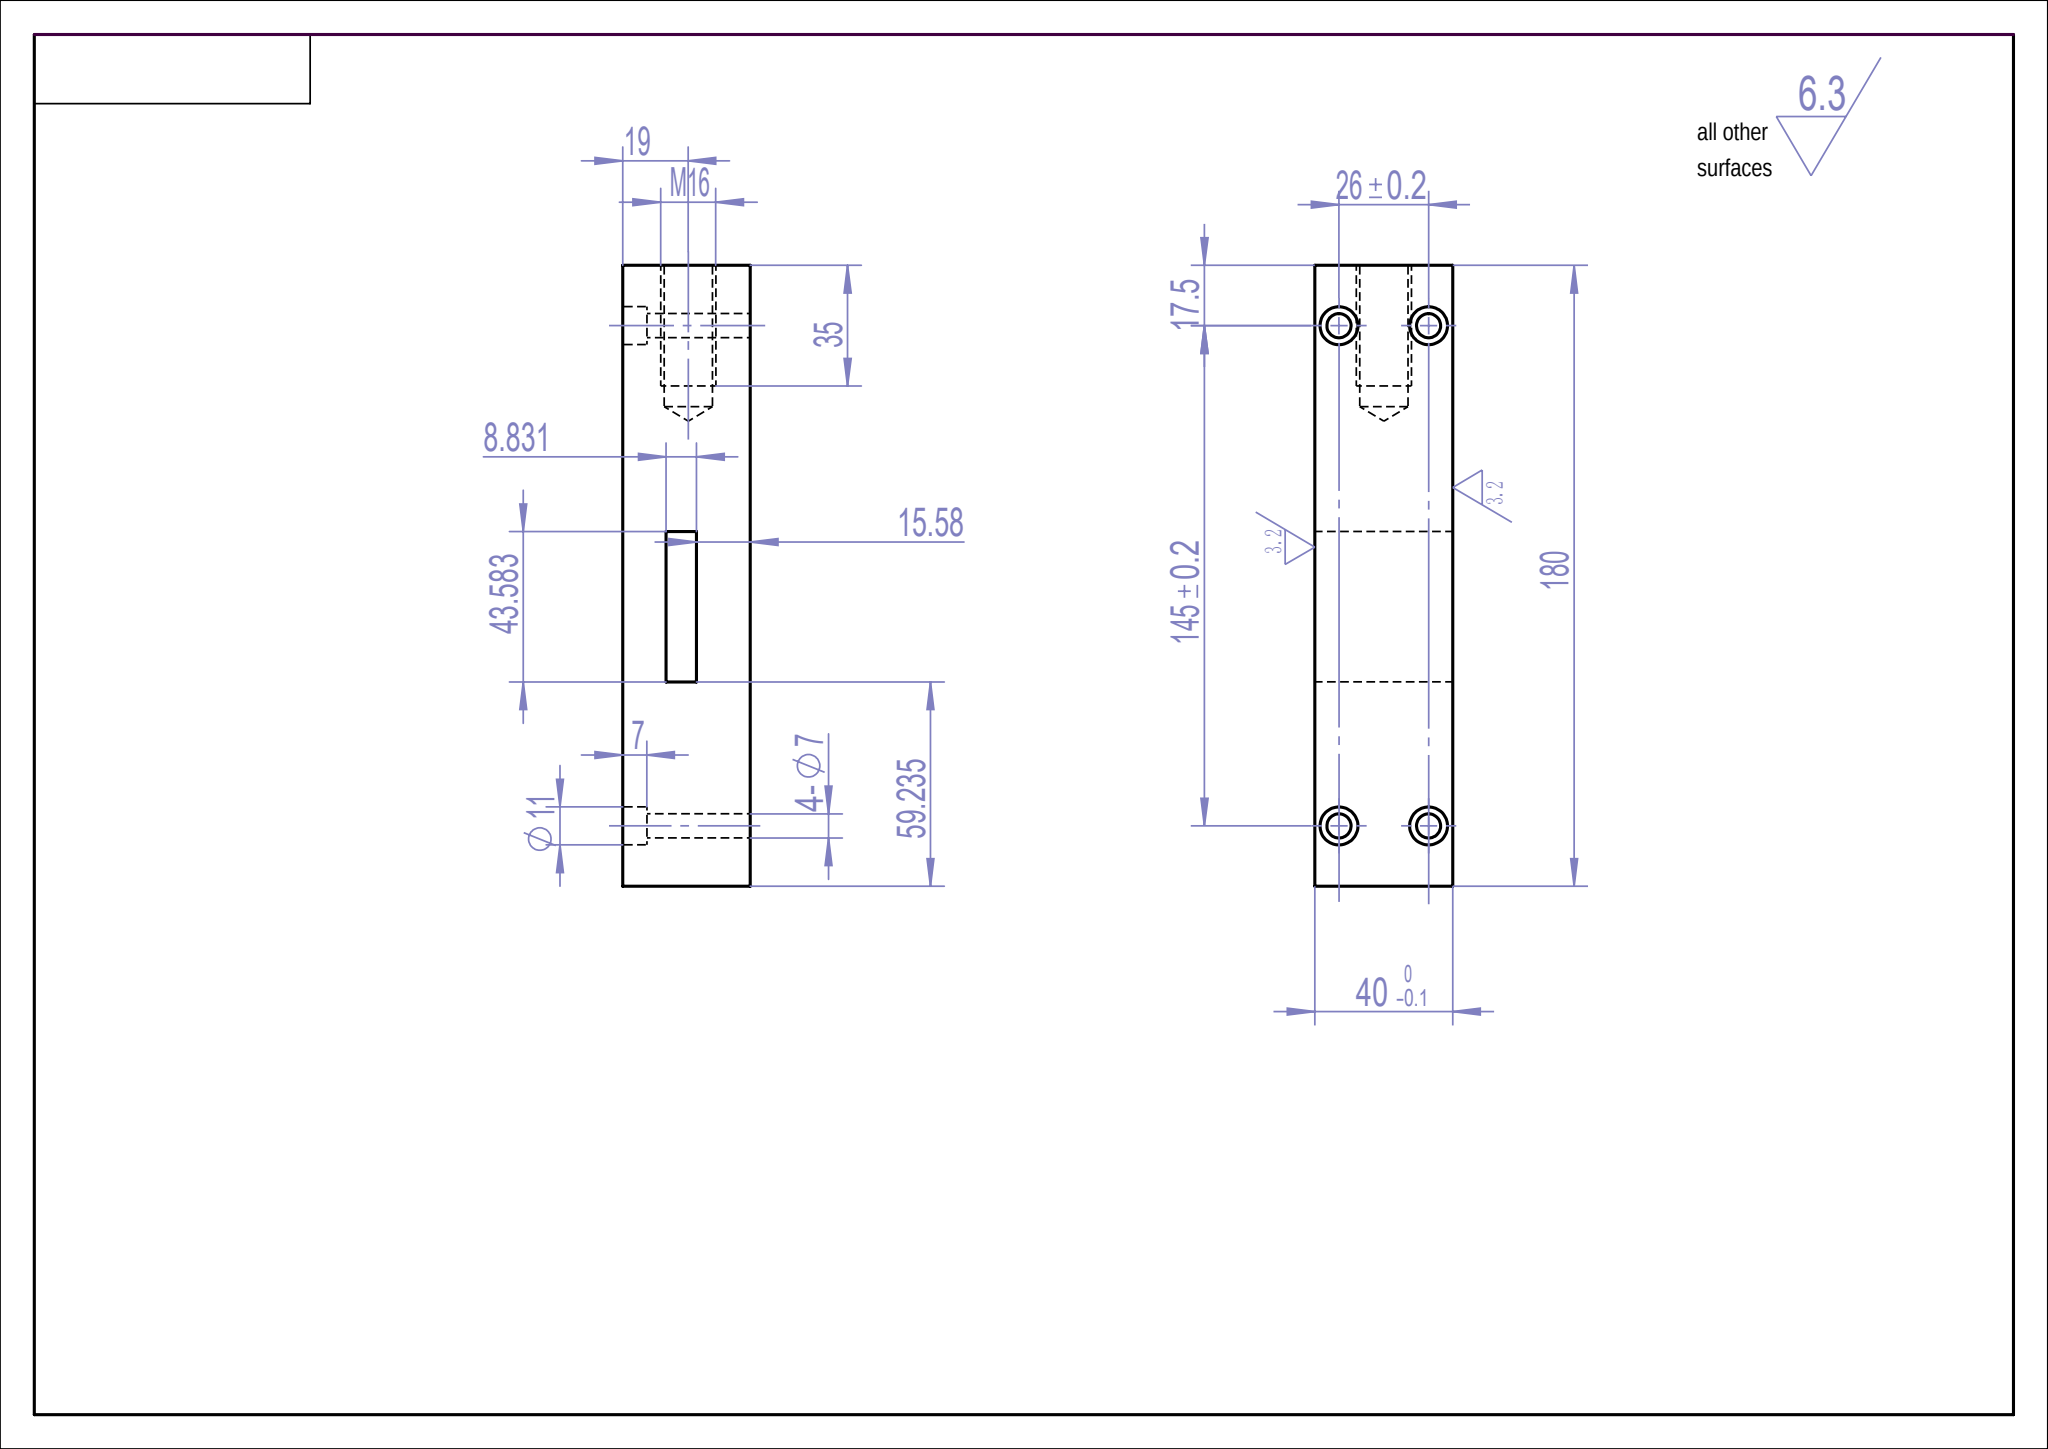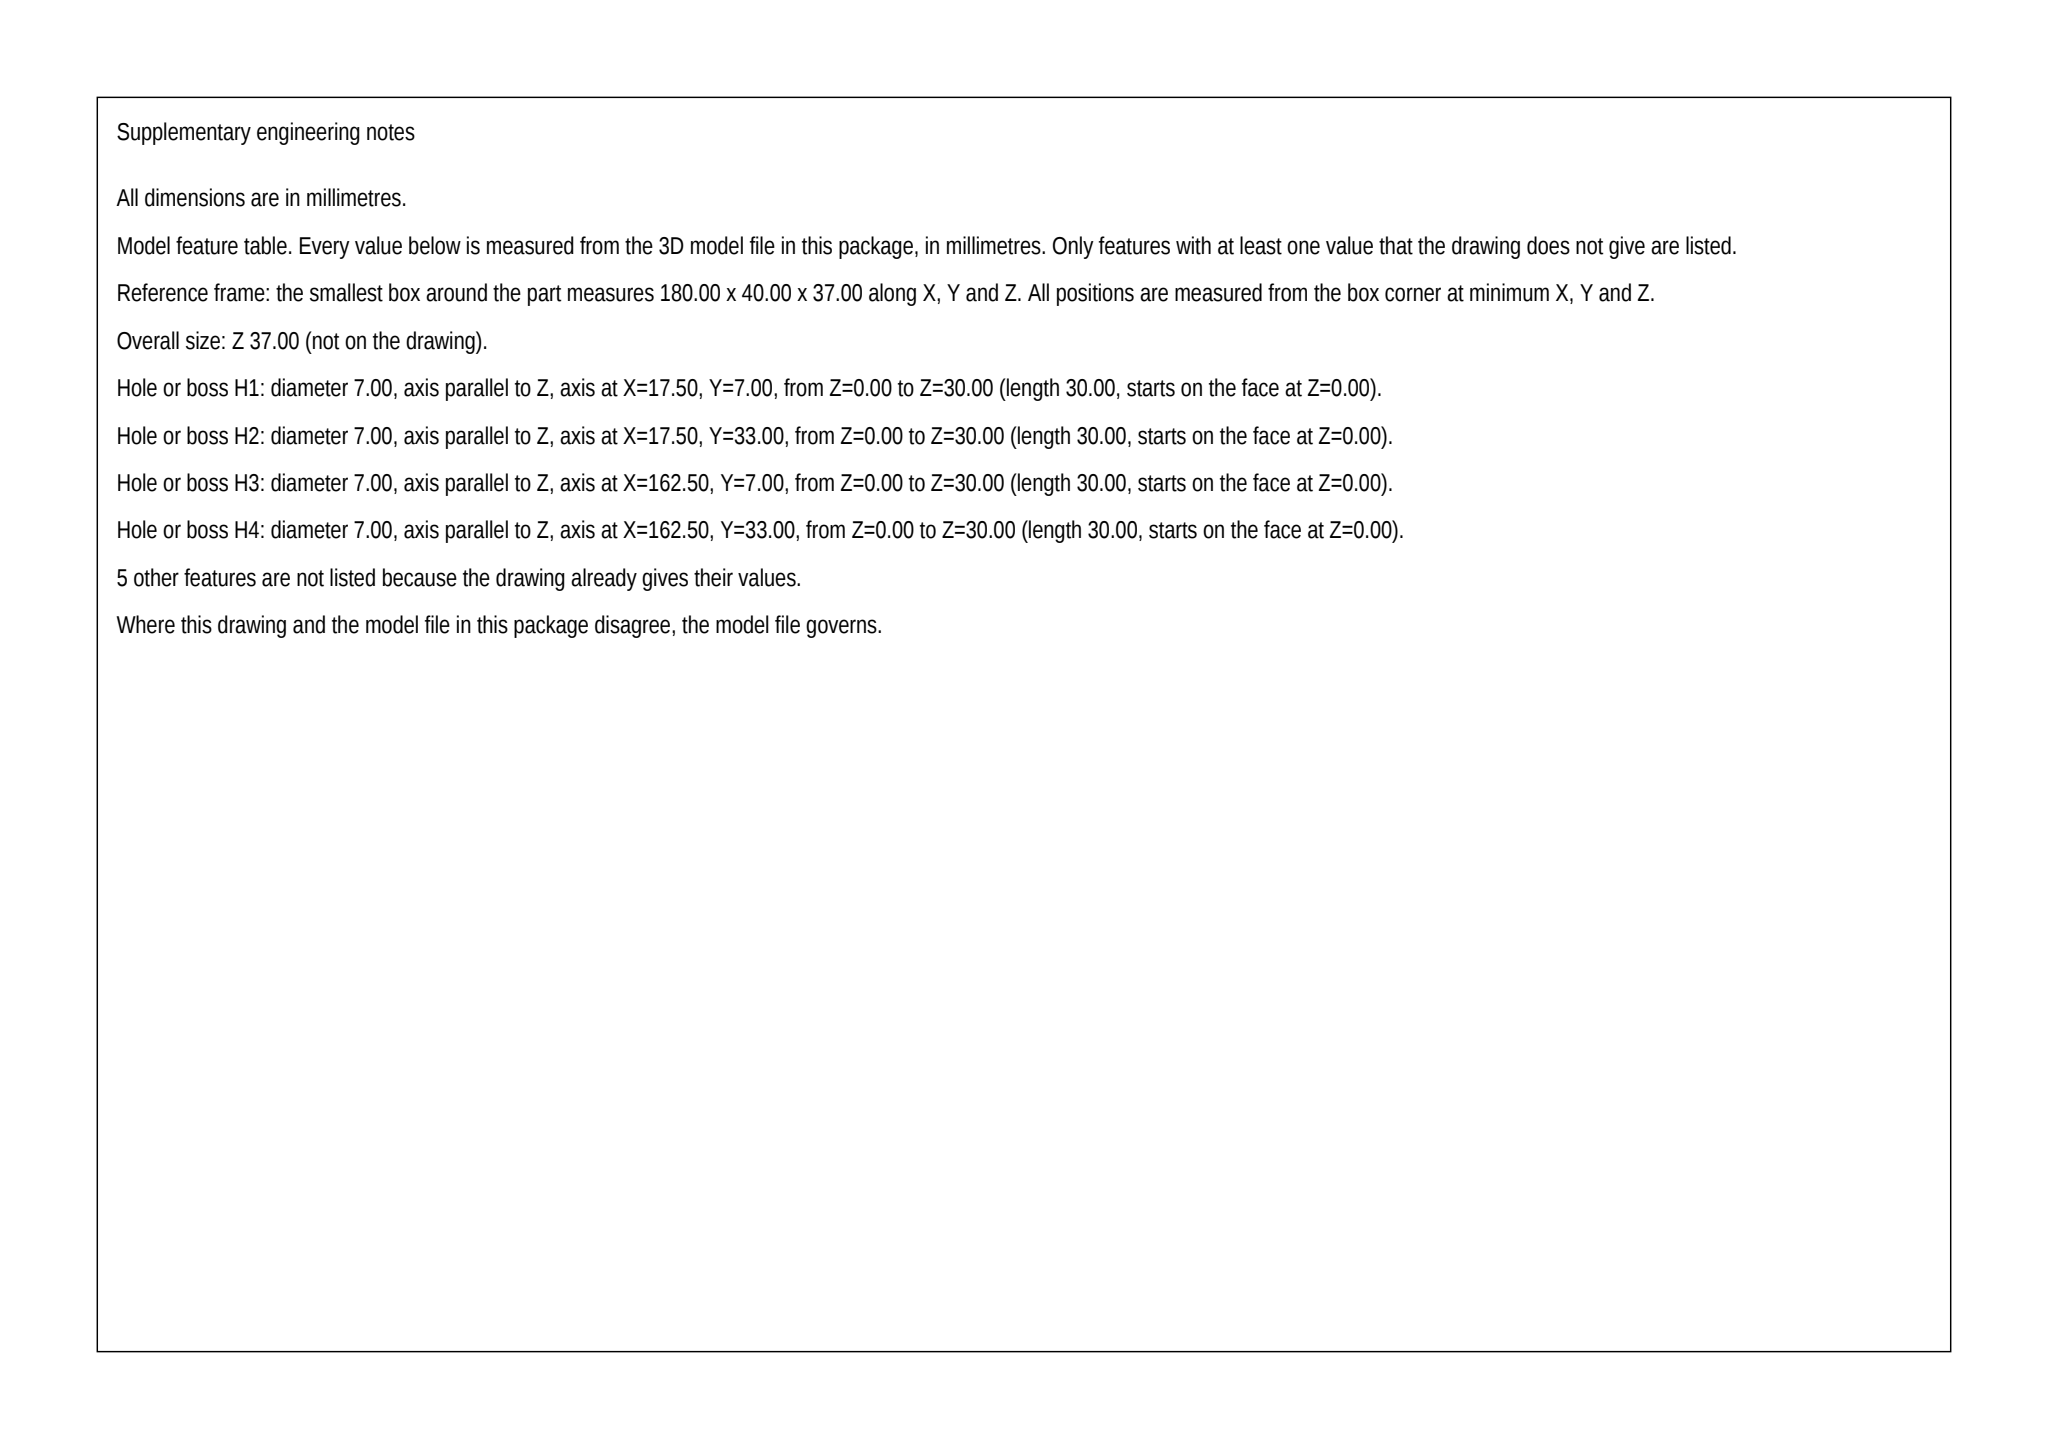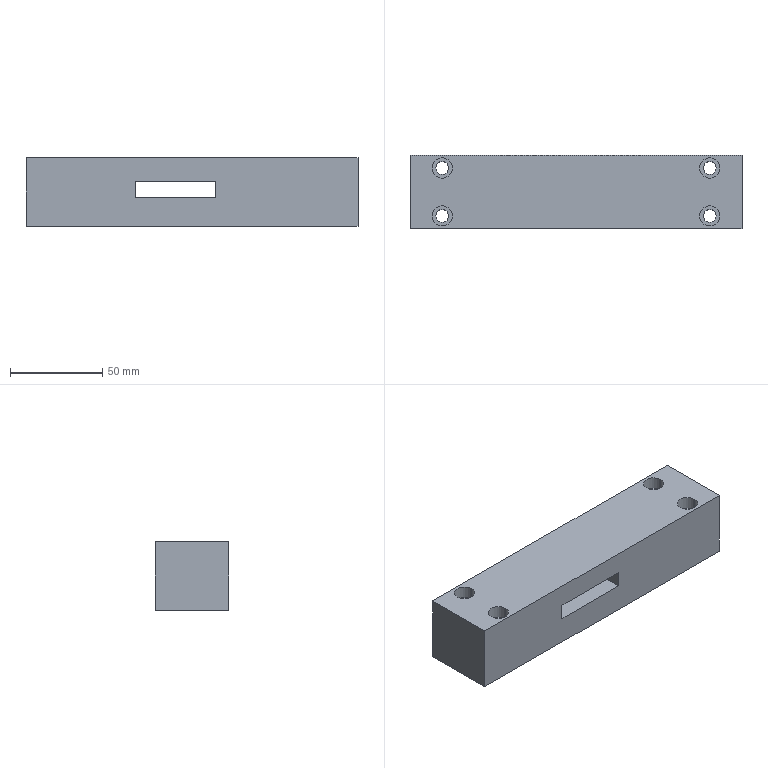Part | SolidWorks | mm | 1 solid | 34 faces | box 180 x 40 x 37 mm | volume 237199 mm3 | cylinder 18 | plane 14 | cone 2 | commonest cylinder face diameters 11 x8 7 x8 14 x2
build123d program:
from build123d import *

# Parameters (mm, degrees)
SKETCH1_W              = 180
SKETCH1_H              = 40
BOSS_EXTRUDE1_DEPTH    = 37
SKETCH2_R              = 5.5
CUT_EXTRUDE1_DEPTH     = 7
SKETCH3_R              = 3.5
CUT_EXTRUDE2_DEPTH     = 37
LPATTERN1_COUNT        = 2
LPATTERN1_PITCH        = 145
LPATTERN1_COUNT_DIR2   = 2
LPATTERN1_PITCH_DIR2   = 26
M16_TAPPED_HOLE1_D     = 14
M16_TAPPED_HOLE1_DEPTH = 41
M16_TAPPED_HOLE1_TIP   = 4.206
SKETCH6_W              = 43.583
SKETCH6_H              = 8.831
CUT_EXTRUDE3_DEPTH     = 78


with BuildPart() as part:
    # Sketch1 → Boss-Extrude1 (new body)
    with BuildSketch(Plane.XY):
        with Locations((11.851, 18.672)):
            Rectangle(SKETCH1_W, SKETCH1_H)
    extrude(amount=BOSS_EXTRUDE1_DEPTH)

    # Sketch2 → Cut-Extrude1 (cut)
    with BuildSketch(Plane.XY.offset(37)):
        with Locations((-60.649, 31.672)):
            Circle(SKETCH2_R)
    cut_extrude1 = extrude(amount=-CUT_EXTRUDE1_DEPTH, mode=Mode.SUBTRACT)

    # Sketch3 → Cut-Extrude2 (cut)
    with BuildSketch(Plane.XY.offset(30)):
        with Locations((-60.649, 31.672)):
            Circle(SKETCH3_R)
    cut_extrude2 = extrude(amount=-CUT_EXTRUDE2_DEPTH, mode=Mode.SUBTRACT)

    # LPattern1: Cut-Extrude1, Cut-Extrude2 2 × 2
    with Locations(*[(i * LPATTERN1_PITCH, -j * LPATTERN1_PITCH_DIR2, 0) for i in range(LPATTERN1_COUNT) for j in range(LPATTERN1_COUNT_DIR2) if (i, j) != (0, 0)]):
        add(cut_extrude1, mode=Mode.SUBTRACT)
        add(cut_extrude2, mode=Mode.SUBTRACT)

    # M16 Tapped Hole1
    with Locations(Plane(origin=(101.851, 18.672, 18), x_dir=(0, 0, 1), z_dir=(1, 0, 0))):
        with Locations((0, 0)):
            Hole(M16_TAPPED_HOLE1_D / 2, depth=M16_TAPPED_HOLE1_DEPTH)
            with Locations((0, 0, -(M16_TAPPED_HOLE1_DEPTH + M16_TAPPED_HOLE1_TIP / 2))):  # 118° drill point
                Cone(0, M16_TAPPED_HOLE1_D / 2, M16_TAPPED_HOLE1_TIP, mode=Mode.SUBTRACT)

    # Sketch6 → Cut-Extrude3 (cut)
    with BuildSketch(Plane.XZ.offset(1.328)):
        with Locations((2.878, 19.996)):
            Rectangle(SKETCH6_W, SKETCH6_H)
    extrude(amount=-CUT_EXTRUDE3_DEPTH, mode=Mode.SUBTRACT)


solid = part.part